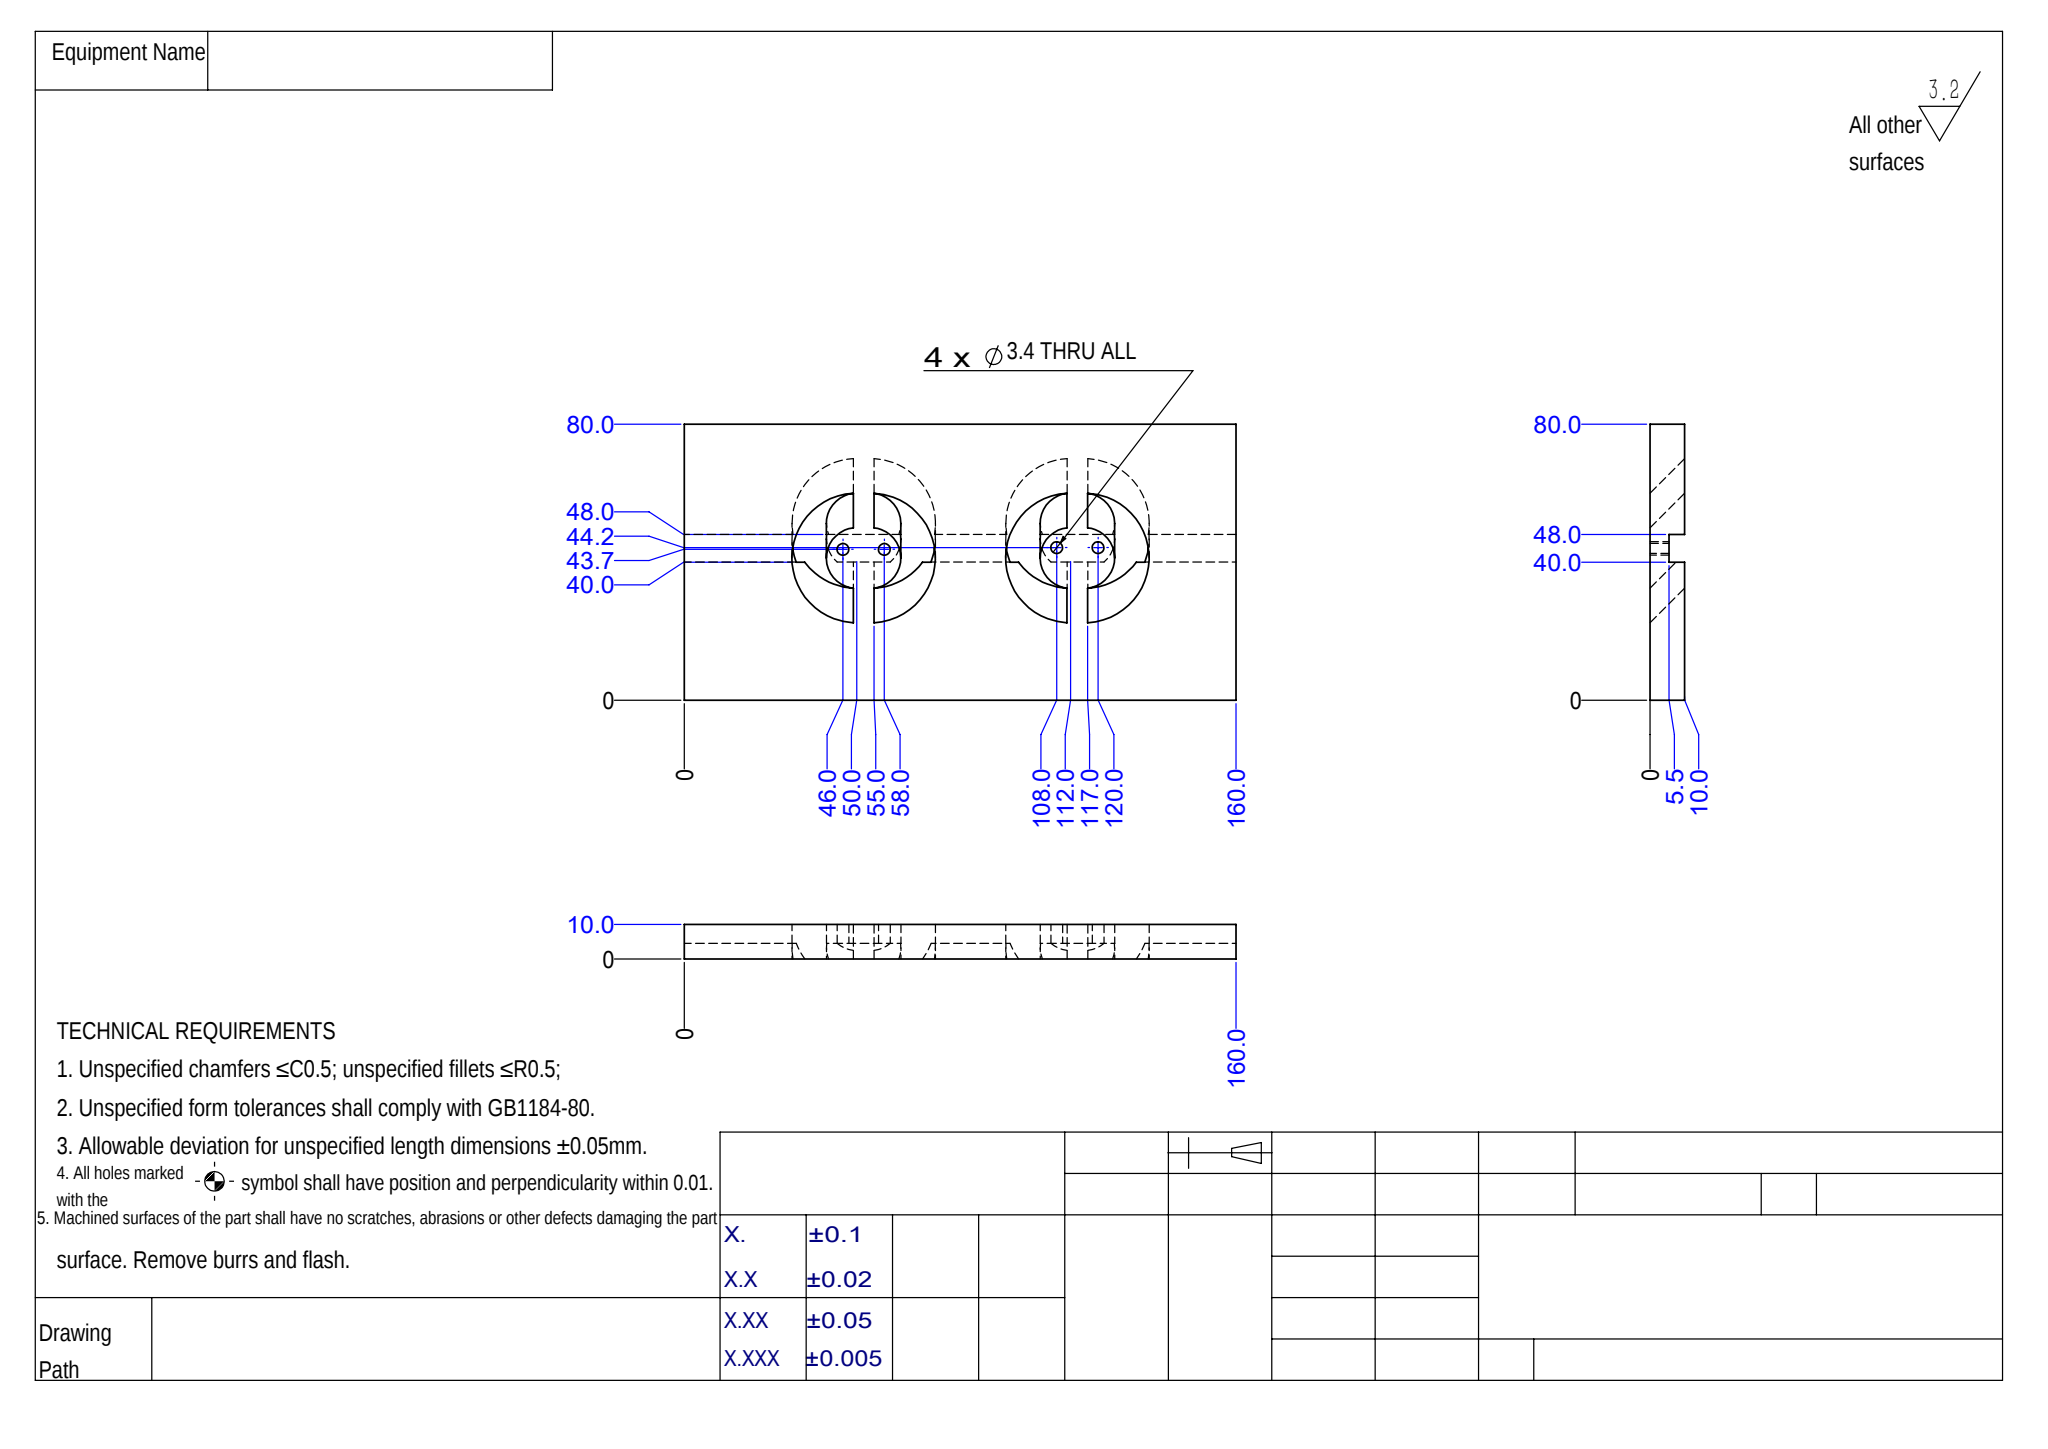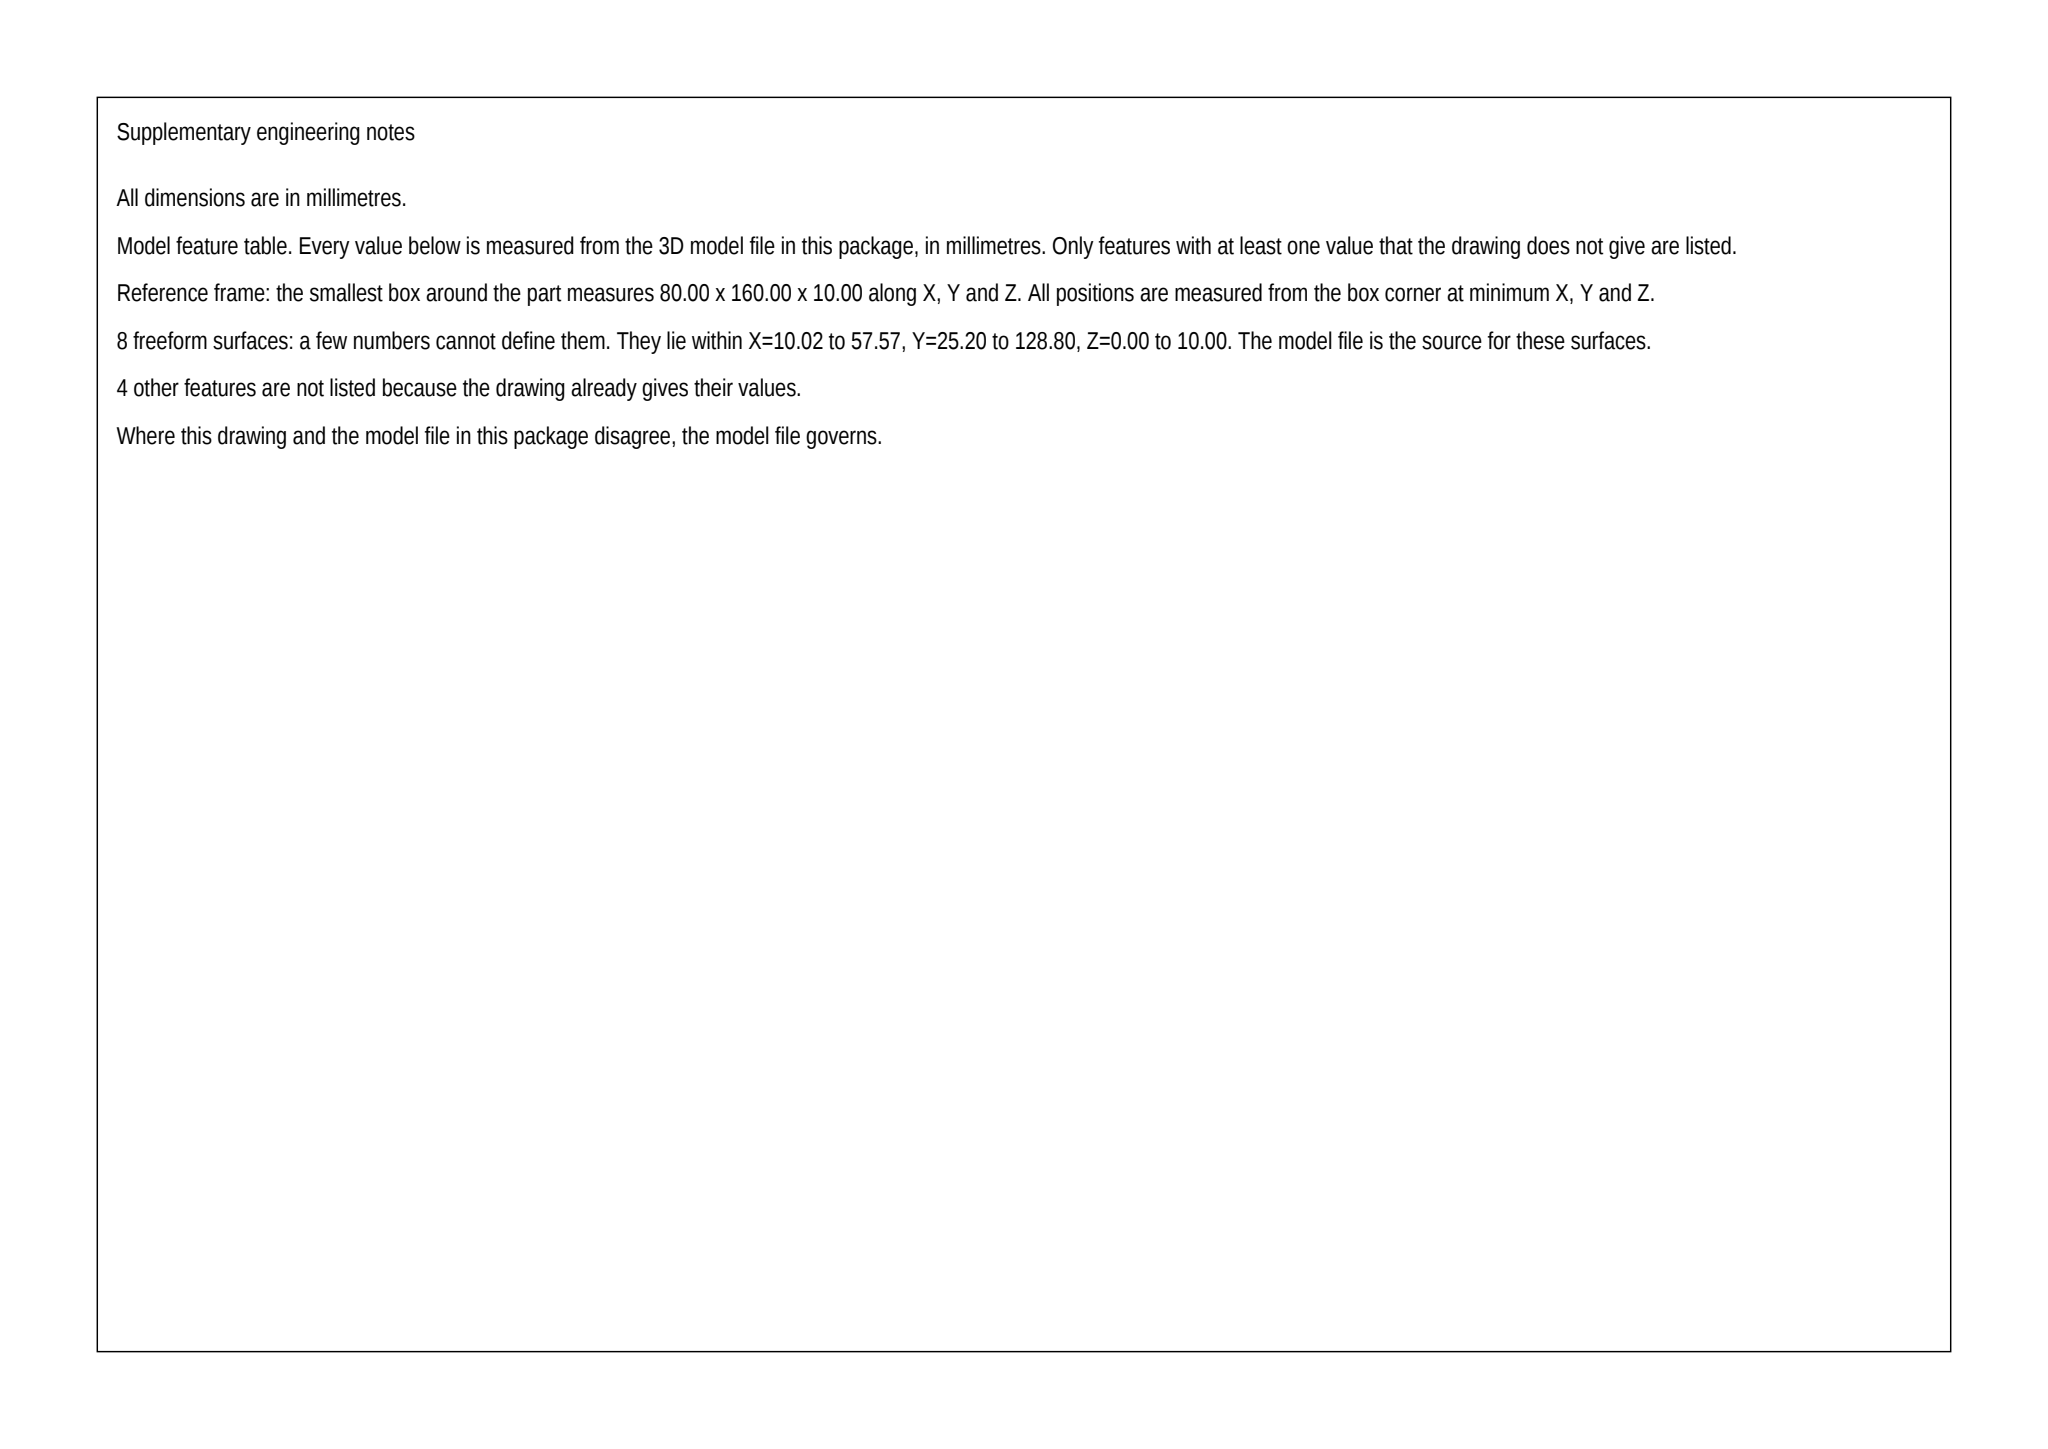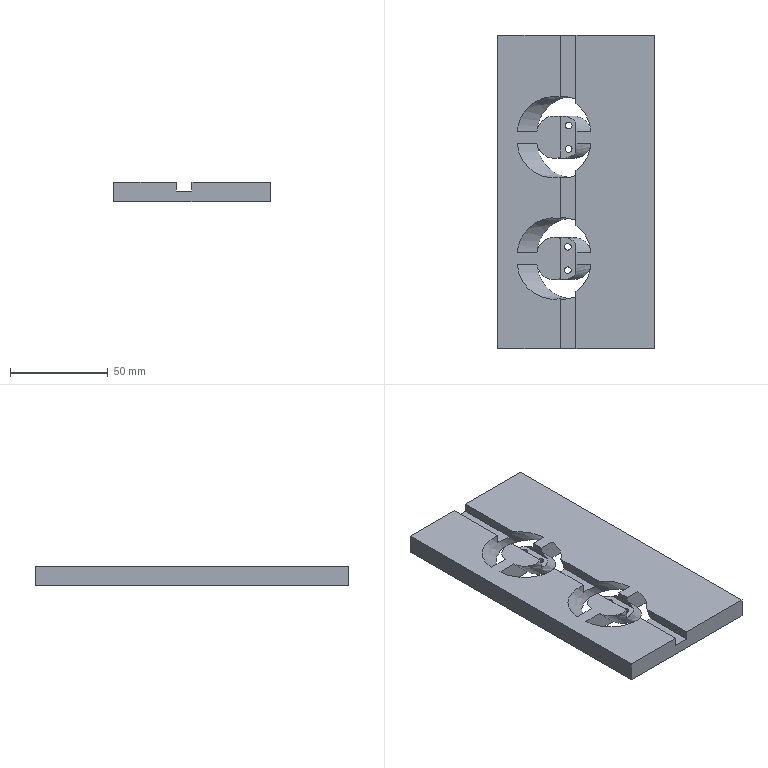Part | SolidWorks | mm | 1 solid | 46 faces | box 80 x 160 x 10 mm | volume 107151 mm3 | plane 30 | cylinder 8 | spline 8 | commonest cylinder face diameters 3.4 x8